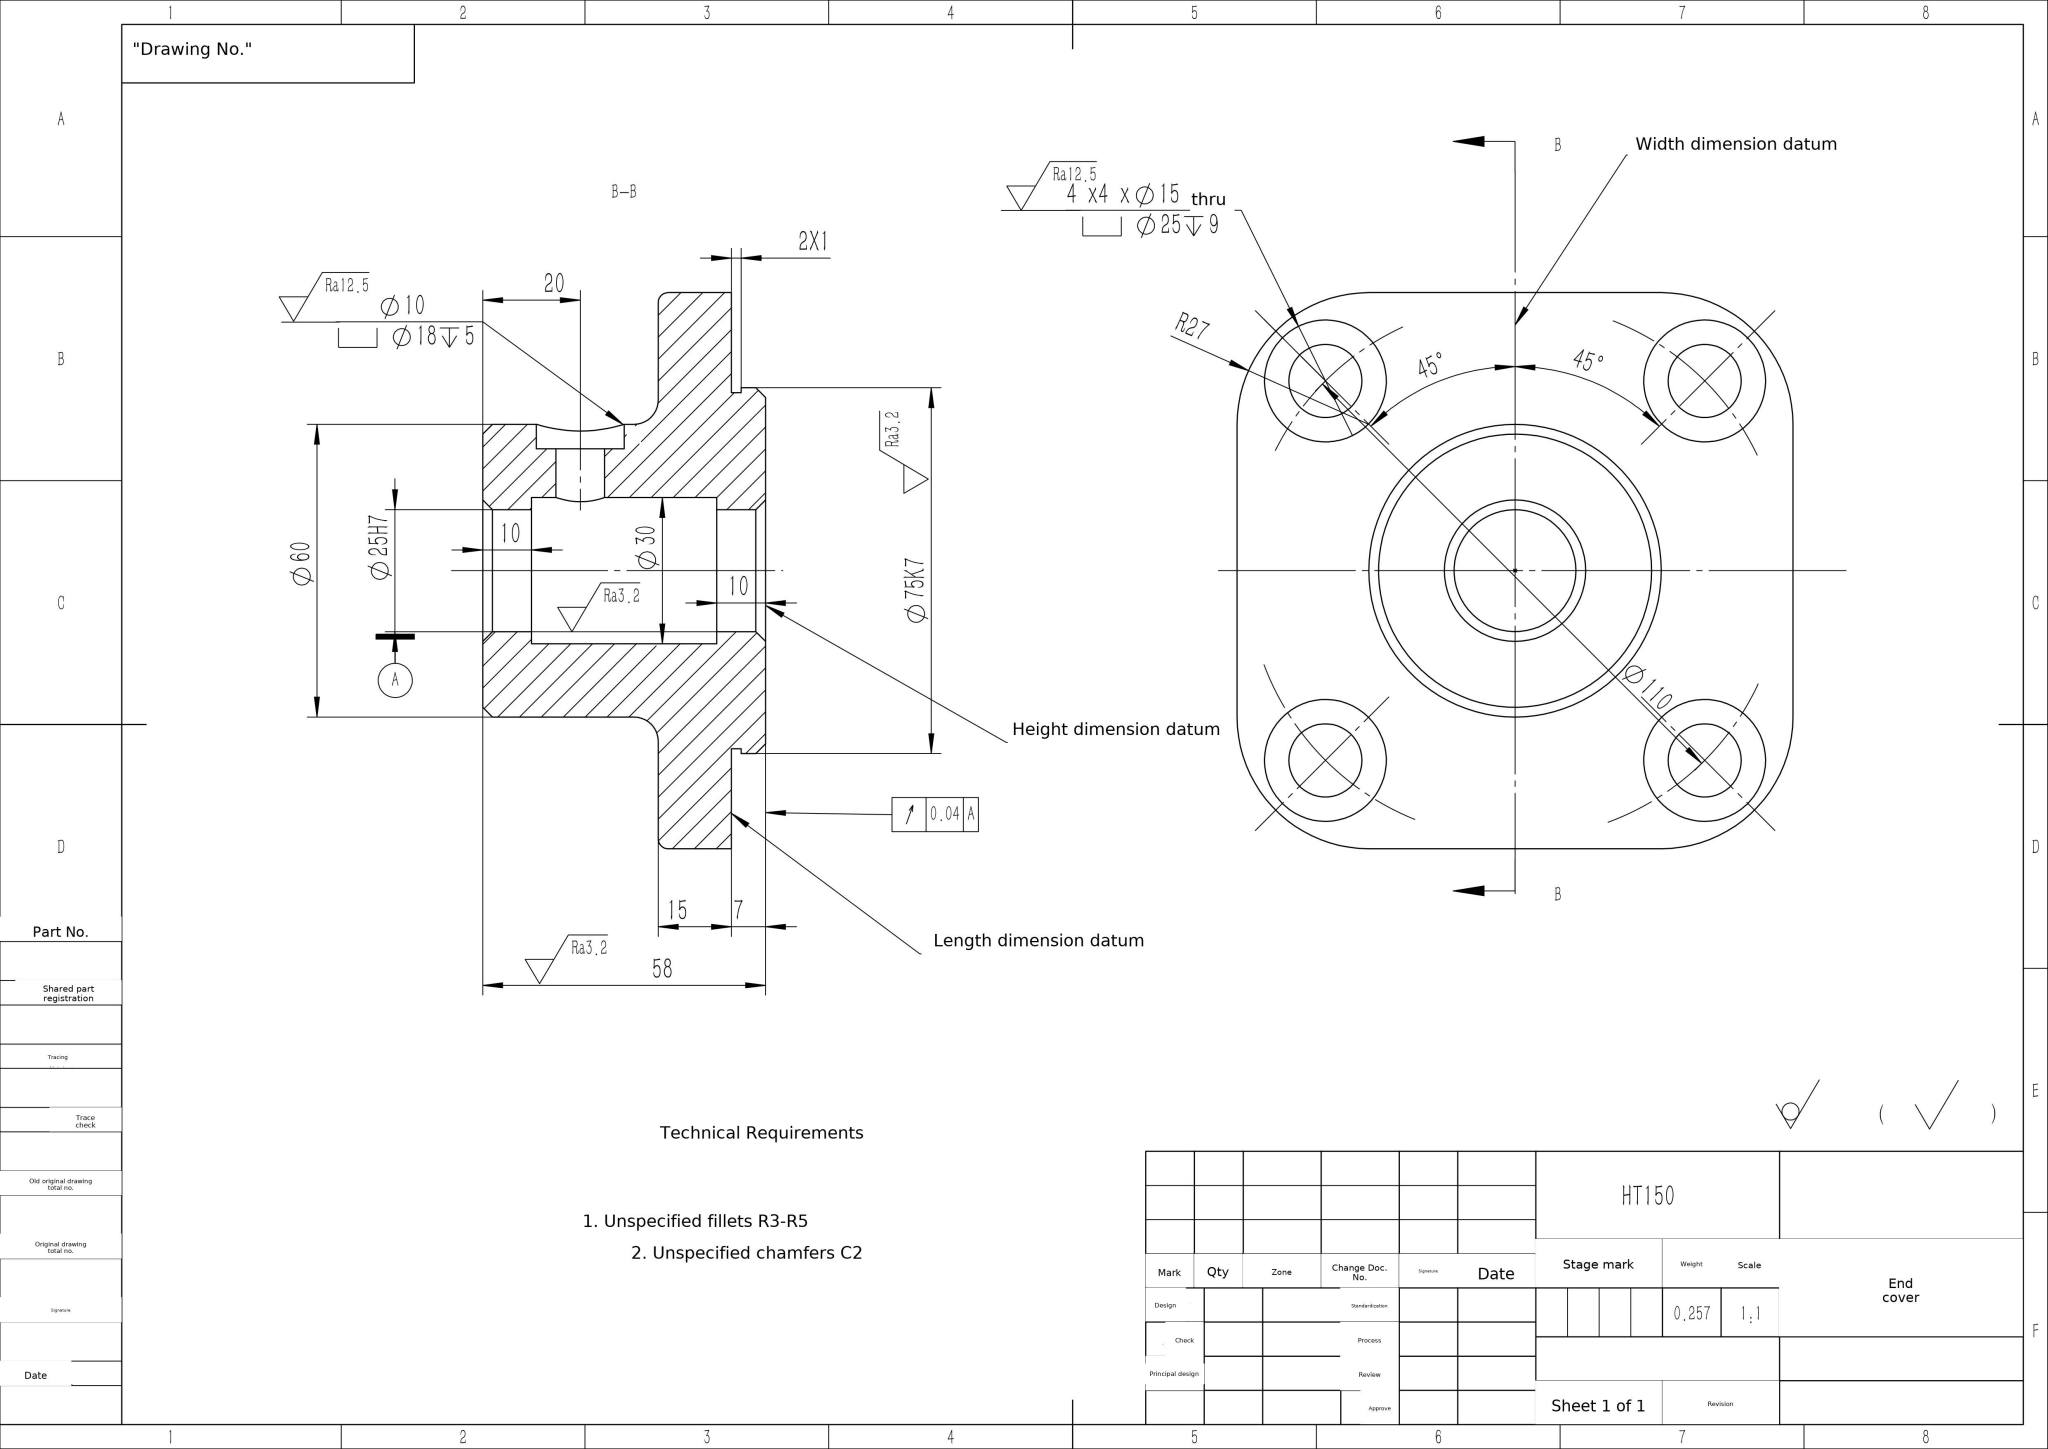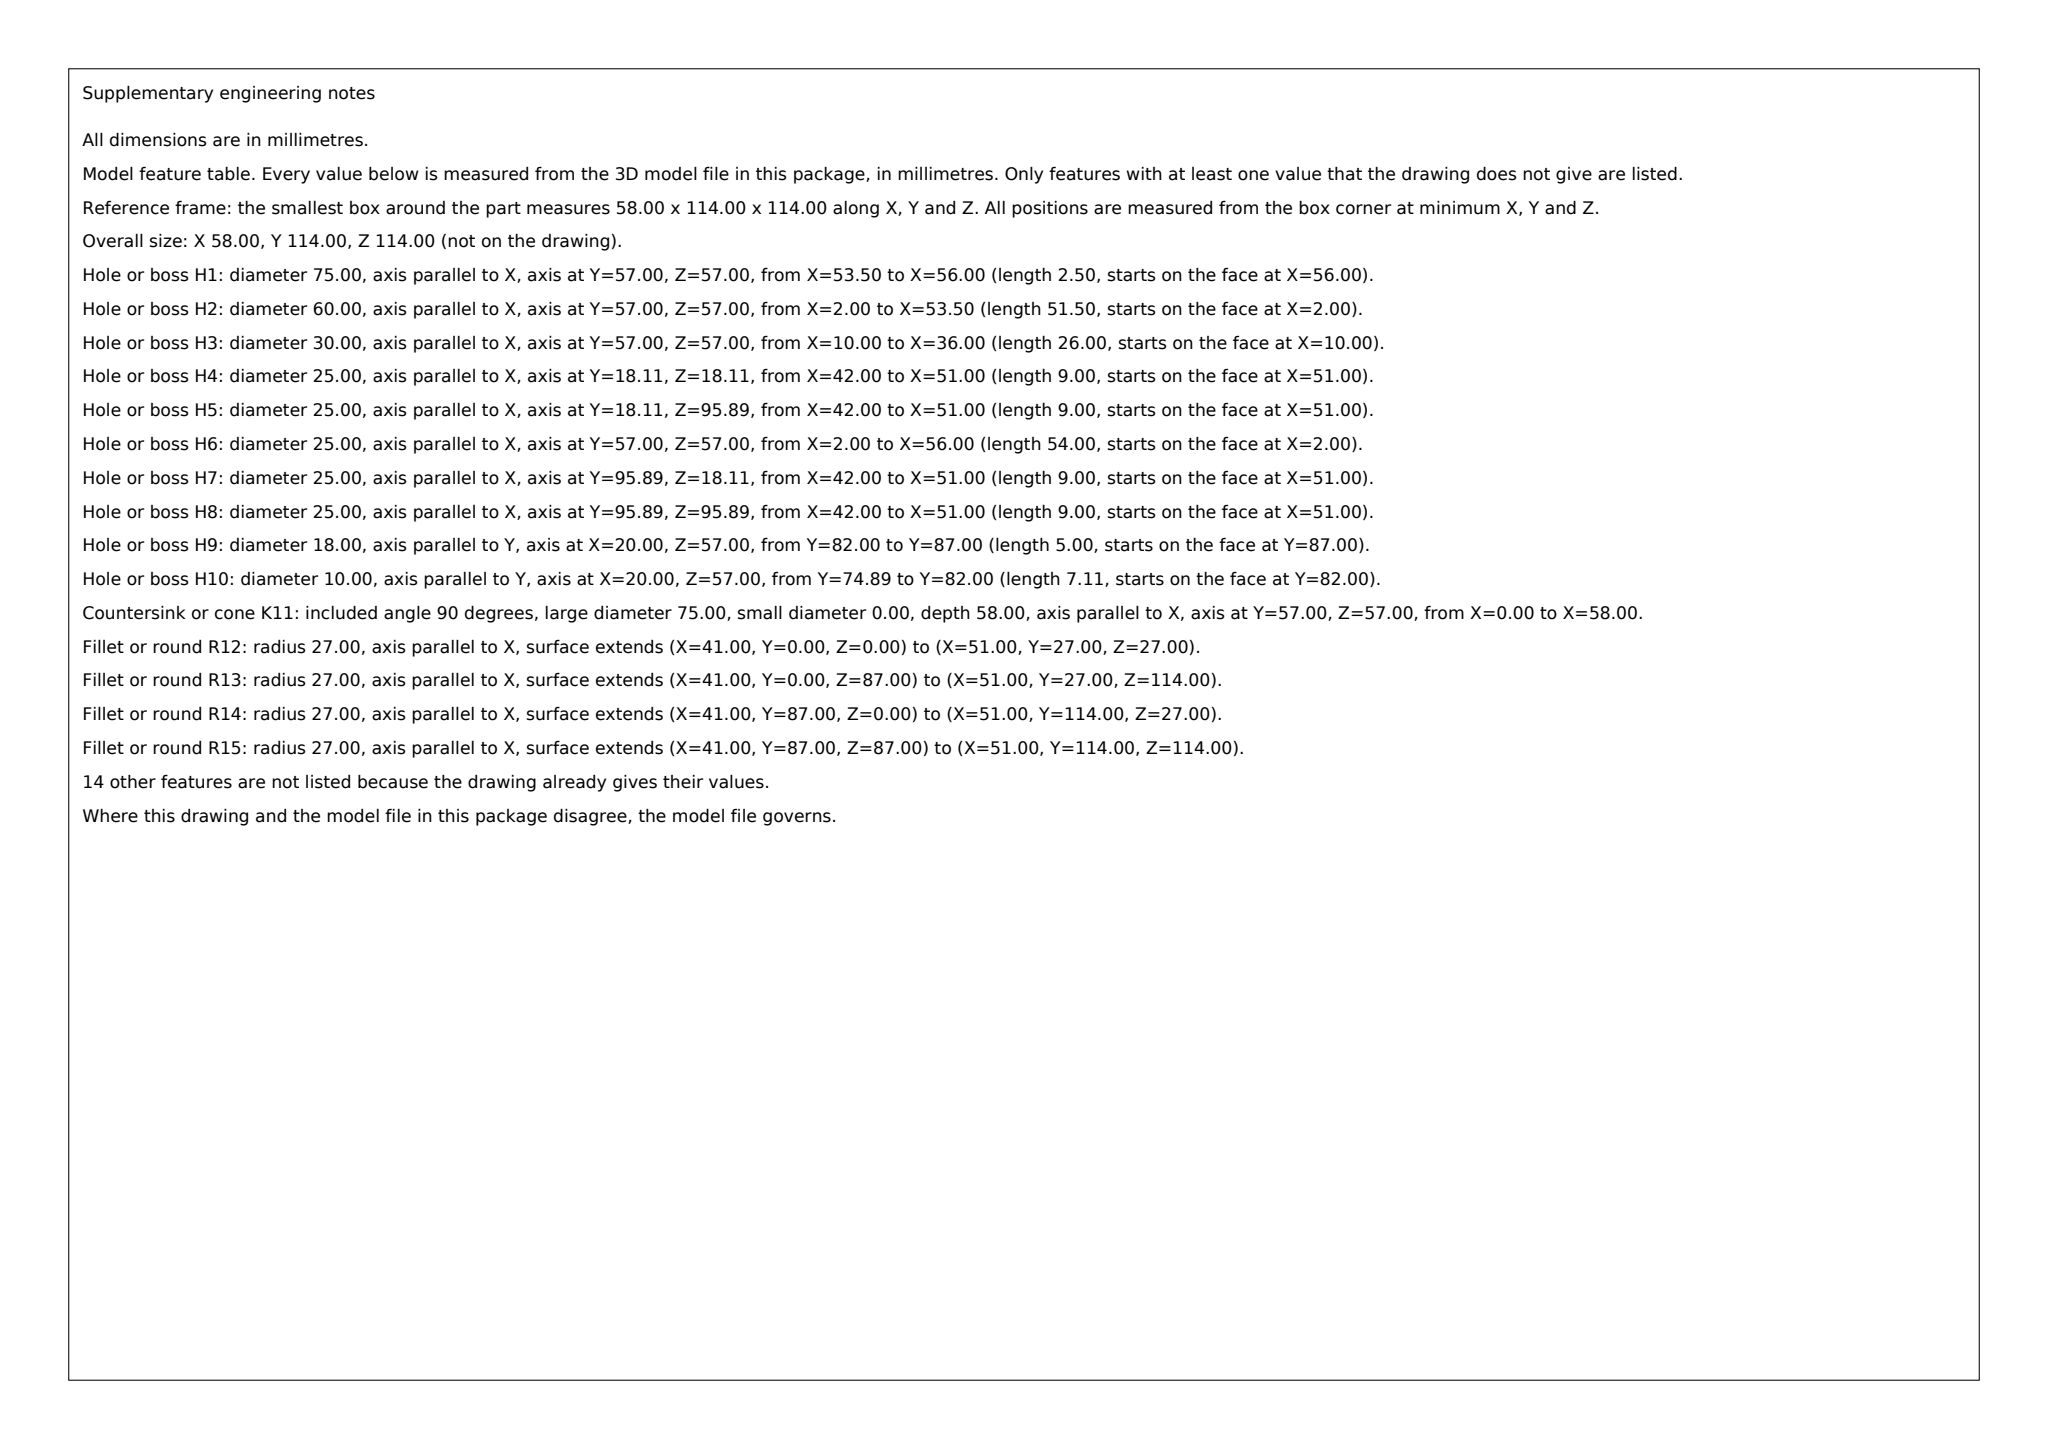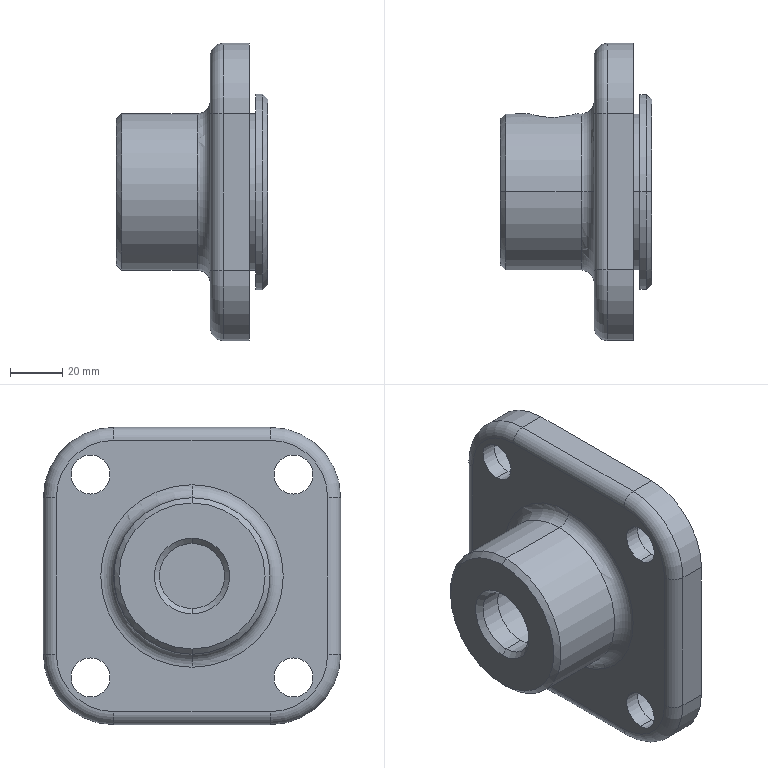Part | SolidWorks | mm | material HT150 | 1 solid | 74 faces | box 58 x 114 x 114 mm | volume 261637 mm3 | cylinder 42 | plane 18 | cone 8 | torus 6 | commonest cylinder face diameters 25 x12 15 x8 10 x6 18 x4 60 x4 54 x4 75 x2 30 x2
build123d program:
from build123d import *

# Parameters (mm, degrees)
SKETCH1_R            = 30
BOSS_EXTRUDE1_DEPTH  = 58
SKETCH2_R            = 37.5
BOSS_EXTRUDE2_DEPTH  = 4.5
BOSS_EXTRUDE3_START  = -7
SKETCH3_R            = 57.5
BOSS_EXTRUDE3_DEPTH  = 15
CHAMFER1_SIZE        = 2
CUT_SWEEP1_PROFILE_R = 5
CUT_SWEEP2_PROFILE_R = 9
SKETCH17_OUTSIDE_W   = 151.534
SKETCH17_OUTSIDE_H   = 151.534
SKETCH17_OUTSIDE_W_2 = 114
SKETCH17_OUTSIDE_H_2 = 114
CUT_EXTRUDE1_DEPTH   = 15
SKETCH18_W           = 114
SKETCH18_H           = 114
BOSS_EXTRUDE4_DEPTH  = 15
FILLET1_R            = 27
SKETCH20_R           = 12.5
CUT_EXTRUDE2_DEPTH   = 9
SKETCH21_R           = 7.5
CUT_EXTRUDE3_DEPTH   = 149
CIRPATTERN1_COUNT    = 4
CHAMFER2_SIZE        = 2
CHAMFER3_SIZE        = 2
FILLET2_R            = 5
FILLET3_R            = 5


with BuildPart() as part:
    # Sketch1 → Boss-Extrude1 (new body)
    with BuildSketch(Plane(origin=(0, 0, 0), x_dir=(0, 0, -1), z_dir=(1, 0, 0))):
        with Locations(Location((0, 0, 0), (0, 0, 180))):
            Circle(SKETCH1_R)
    extrude(amount=BOSS_EXTRUDE1_DEPTH)

    # Sketch2 → Boss-Extrude2 (add)
    with BuildSketch(Plane(origin=(58, 0, 0), x_dir=(0, 0, -1), z_dir=(1, 0, 0))):
        Circle(SKETCH2_R)
    extrude(amount=-BOSS_EXTRUDE2_DEPTH)

    # Sketch3 → Boss-Extrude3 (add)
    with BuildSketch(Plane(origin=(58, 0, 0), x_dir=(0, 0, -1), z_dir=(1, 0, 0)).offset(BOSS_EXTRUDE3_START)):
        Circle(SKETCH3_R)
    extrude(amount=-BOSS_EXTRUDE3_DEPTH)

    # Sketch4 → Cut-Revolve1 (revolve, cut)
    with BuildSketch(Plane.XY, mode=Mode.PRIVATE) as cut_revolve1_sk:
        Polygon((0, 12.5), (10, 12.5), (10, 15), (48, 15), (48, 12.5), (58, 12.5), (58, 0), (0, 0), align=None)
    revolve(cut_revolve1_sk.sketch.rotate(Axis((58, 0, 0), (-1, 0, 0)), 90), axis=Axis((58, 0, 0), (-1, 0, 0)), mode=Mode.SUBTRACT)

    # Chamfer1
    chamfer1_edges = [part.edges().sort_by_distance(p)[0] for p in [
        (0, 0, 12.5),
        (58, 0, 12.5),
    ]]
    chamfer(chamfer1_edges, length=CHAMFER1_SIZE)

    # Cut-Sweep1: sweep along a path in Sketch5
    with BuildLine(Plane.XY) as cut_sweep1_path:
        Line((20, 32.658), (20, 17.892))
    # Cut-Sweep1 profile (on start of the path) → Cut-Sweep1 (sweep, cut)
    with BuildSketch(Plane(origin=(20, 32.658, 0), x_dir=(-1, 0, 0), z_dir=(0, -1, 0))):
        Circle(CUT_SWEEP1_PROFILE_R)
    sweep(path=cut_sweep1_path.line, mode=Mode.SUBTRACT)

    # Cut-Sweep2: sweep along a path in Sketch10
    with BuildLine(Plane.XY) as cut_sweep2_path:
        Line((20, 25), (20, 29.58))
        Line((20, 29.58), (20, 30))
    # Cut-Sweep2 profile (on start of the path) → Cut-Sweep2 (sweep, cut)
    with BuildSketch(Plane(origin=(20, 25, 0), x_dir=(1, 0, 0), z_dir=(0, 1, 0))):
        Circle(CUT_SWEEP2_PROFILE_R)
    sweep(path=cut_sweep2_path.line, mode=Mode.SUBTRACT)

    # Sketch17 outside → Cut-Extrude1 (cut)
    with BuildSketch(Plane(origin=(51, 0, 0), x_dir=(0, 0, -1), z_dir=(1, 0, 0))):
        Rectangle(SKETCH17_OUTSIDE_W, SKETCH17_OUTSIDE_H)
        Rectangle(SKETCH17_OUTSIDE_W_2, SKETCH17_OUTSIDE_H_2, mode=Mode.SUBTRACT)
    extrude(amount=-CUT_EXTRUDE1_DEPTH, mode=Mode.SUBTRACT)

    # Sketch18 → Boss-Extrude4 (add)
    with BuildSketch(Plane(origin=(51, 0, 0), x_dir=(0, 0, -1), z_dir=(1, 0, 0))):
        Rectangle(SKETCH18_W, SKETCH18_H)
    extrude(amount=-BOSS_EXTRUDE4_DEPTH)

    # Fillet1
    fillet1_edges = [part.edges().sort_by_distance(p)[0] for p in [
        (43.5, -57, 57),
        (43.5, 57, -57),
        (43.5, -57, -57),
        (43.5, 57, 57),
    ]]
    fillet(fillet1_edges, radius=FILLET1_R)

    # Sketch20 → Cut-Extrude2 (cut)
    with BuildSketch(Plane(origin=(51, 0, 0), x_dir=(0, 0, -1), z_dir=(1, 0, 0))):
        with Locations((-38.891, 38.891)):
            Circle(SKETCH20_R)
    cut_extrude2 = extrude(amount=-CUT_EXTRUDE2_DEPTH, mode=Mode.SUBTRACT)

    # Sketch21 → Cut-Extrude3 (cut)
    with BuildSketch(Plane(origin=(42, 0, 0), x_dir=(0, 0, -1), z_dir=(1, 0, 0))):
        with Locations((-38.891, 38.891)):
            Circle(SKETCH21_R)
    cut_extrude3 = extrude(amount=-CUT_EXTRUDE3_DEPTH, mode=Mode.SUBTRACT)

    # CirPattern1: Cut-Extrude2, Cut-Extrude3 ×4 about axis
    cirpattern1_axis = Axis((0, 0, 0), (1, 0, 0))
    add([cut_extrude2.rotate(cirpattern1_axis, i * 360 / CIRPATTERN1_COUNT) for i in range(1, CIRPATTERN1_COUNT)], mode=Mode.SUBTRACT)
    add([cut_extrude3.rotate(cirpattern1_axis, i * 360 / CIRPATTERN1_COUNT) for i in range(1, CIRPATTERN1_COUNT)], mode=Mode.SUBTRACT)

    # Chamfer2
    chamfer2_edges = [part.edges().sort_by_distance(p)[0] for p in [
        (58, 0, 37.5),
    ]]
    chamfer(chamfer2_edges, length=CHAMFER2_SIZE)

    # Chamfer3
    chamfer3_edges = [part.edges().sort_by_distance(p)[0] for p in [
        (0, 0, -30),
    ]]
    chamfer(chamfer3_edges, length=CHAMFER3_SIZE)

    # Fillet2
    fillet2_edges = [part.edges().sort_by_distance(p)[0] for p in [
        (36, 0, -57),
        (36, 57, 0),
        (36, -57, 0),
        (36, 0, 57),
        (36, -49.092, 49.092),
        (36, -49.092, -49.092),
        (36, 49.092, 49.092),
        (36, 49.092, -49.092),
    ]]
    fillet(fillet2_edges, radius=FILLET2_R)

    # Fillet3
    fillet3_edges = [part.edges().sort_by_distance(p)[0] for p in [
        (36, 0, -30),
    ]]
    fillet(fillet3_edges, radius=FILLET3_R)


solid = part.part